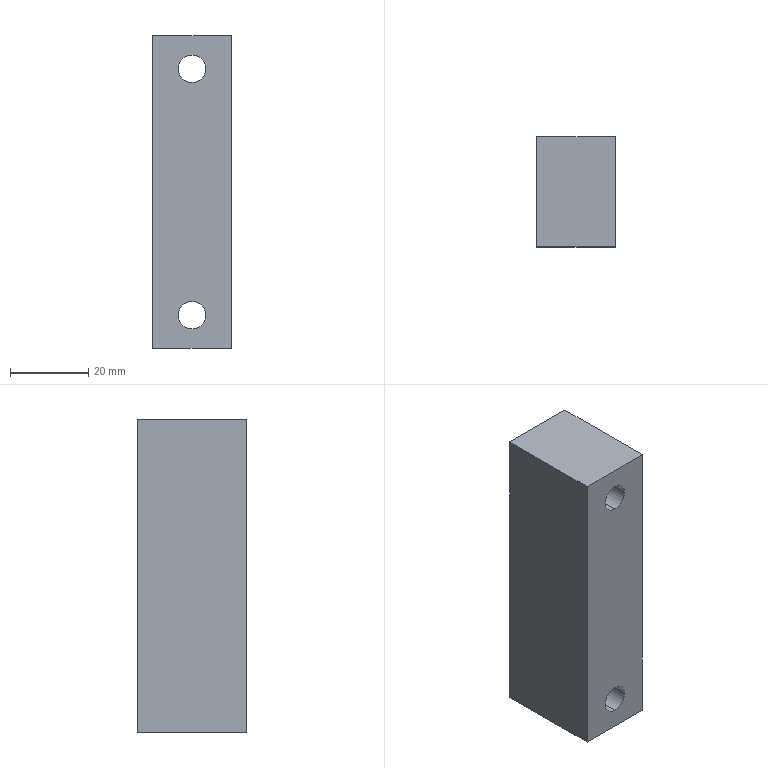Component | SolidWorks | BearingHeighteningSeat-1 | 1 solid | 10 faces | box 20 x 28 x 80 mm | volume 42645 mm3 | plane 6 | cylinder 4 | commonest cylinder face diameters 7 x4
build123d program:
from build123d import *

# Parameters (mm, degrees)
SKETCH1_W      = 80
SKETCH1_H      = 20
SKETCH1_R      = 3.5
EXTRUDE1_DEPTH = 28


with BuildPart() as part:
    # Sketch1 → Extrude1 (new body)
    with BuildSketch(Plane.XY):
        with Locations((-20.645, 10.76)):
            Rectangle(SKETCH1_W, SKETCH1_H)
        with Locations((-52.145, 10.76)):
            Circle(SKETCH1_R, mode=Mode.SUBTRACT)
        with Locations((10.855, 10.76)):
            Circle(SKETCH1_R, mode=Mode.SUBTRACT)
    extrude(amount=EXTRUDE1_DEPTH)


solid = part.part

# Placed as in the assembly
solid = solid.moved(Location((190.976, 153.983, 79.382), (90, 0, 90)))
STEP:
#1=COLOUR_RGB('',0.7922,0.8196,0.9333);
#2=FILL_AREA_STYLE_COLOUR('',#1);
#3=FILL_AREA_STYLE('',(#2));
#4=SURFACE_STYLE_FILL_AREA(#3);
#5=SURFACE_SIDE_STYLE('',(#4));
#6=SURFACE_STYLE_USAGE(.BOTH.,#5);
#7=PRESENTATION_STYLE_ASSIGNMENT((#6));
#8=CARTESIAN_POINT('',(7.095,6.062,3.415));
#9=VERTEX_POINT('',#8);
#10=CARTESIAN_POINT('',(7.095,6.062,3.69));
#11=VERTEX_POINT('',#10);
#12=CARTESIAN_POINT('',(7.095,6.062,3.553));
#13=DIRECTION('',(-0.,1.,-0.));
#14=DIRECTION('',(0.,0.,1.));
#15=AXIS2_PLACEMENT_3D('',#12,#13,#14);
#16=CIRCLE('',#15,0.1378);
#17=EDGE_CURVE('',#9,#11,#16,.T.);
#18=ORIENTED_EDGE('',*,*,#17,.T.);
#19=CARTESIAN_POINT('',(7.095,4.96,3.69));
#20=VERTEX_POINT('',#19);
#21=CARTESIAN_POINT('',(7.095,6.062,3.69));
#22=DIRECTION('',(0.,-1.,0.));
#23=VECTOR('',#22,39.37);
#24=LINE('',#21,#23);
#25=EDGE_CURVE('',#11,#20,#24,.T.);
#26=ORIENTED_EDGE('',*,*,#25,.T.);
#27=CARTESIAN_POINT('',(7.095,4.96,3.415));
#28=VERTEX_POINT('',#27);
#29=CARTESIAN_POINT('',(7.095,4.96,3.553));
#30=DIRECTION('',(-0.,1.,-0.));
#31=DIRECTION('',(0.,0.,1.));
#32=AXIS2_PLACEMENT_3D('',#29,#30,#31);
#33=CIRCLE('',#32,0.1378);
#34=EDGE_CURVE('',#28,#20,#33,.T.);
#35=ORIENTED_EDGE('',*,*,#34,.F.);
#36=CARTESIAN_POINT('',(7.095,6.062,3.415));
#37=DIRECTION('',(0.,-1.,0.));
#38=VECTOR('',#37,39.37);
#39=LINE('',#36,#38);
#40=EDGE_CURVE('',#9,#28,#39,.T.);
#41=ORIENTED_EDGE('',*,*,#40,.F.);
#42=EDGE_LOOP('',(#18,#26,#35,#41));
#43=FACE_OUTER_BOUND('',#42,.T.);
#44=CARTESIAN_POINT('',(7.095,6.062,3.553));
#45=DIRECTION('',(0.,-1.,0.));
#46=DIRECTION('',(0.,0.,-1.));
#47=AXIS2_PLACEMENT_3D('',#44,#45,#46);
#48=CYLINDRICAL_SURFACE('',#47,0.1378);
#49=ADVANCED_FACE('',(#43),#48,.F.);
#50=CARTESIAN_POINT('',(7.095,6.062,0.9345));
#51=VERTEX_POINT('',#50);
#52=CARTESIAN_POINT('',(7.095,6.062,1.21));
#53=VERTEX_POINT('',#52);
#54=CARTESIAN_POINT('',(7.095,6.062,1.072));
#55=DIRECTION('',(-0.,1.,-0.));
#56=DIRECTION('',(0.,0.,1.));
#57=AXIS2_PLACEMENT_3D('',#54,#55,#56);
#58=CIRCLE('',#57,0.1378);
#59=EDGE_CURVE('',#51,#53,#58,.T.);
#60=ORIENTED_EDGE('',*,*,#59,.T.);
#61=CARTESIAN_POINT('',(7.095,4.96,1.21));
#62=VERTEX_POINT('',#61);
#63=CARTESIAN_POINT('',(7.095,6.062,1.21));
#64=DIRECTION('',(0.,-1.,0.));
#65=VECTOR('',#64,39.37);
#66=LINE('',#63,#65);
#67=EDGE_CURVE('',#53,#62,#66,.T.);
#68=ORIENTED_EDGE('',*,*,#67,.T.);
#69=CARTESIAN_POINT('',(7.095,4.96,0.9345));
#70=VERTEX_POINT('',#69);
#71=CARTESIAN_POINT('',(7.095,4.96,1.072));
#72=DIRECTION('',(-0.,1.,-0.));
#73=DIRECTION('',(0.,0.,1.));
#74=AXIS2_PLACEMENT_3D('',#71,#72,#73);
#75=CIRCLE('',#74,0.1378);
#76=EDGE_CURVE('',#70,#62,#75,.T.);
#77=ORIENTED_EDGE('',*,*,#76,.F.);
#78=CARTESIAN_POINT('',(7.095,6.062,0.9345));
#79=DIRECTION('',(0.,-1.,0.));
#80=VECTOR('',#79,39.37);
#81=LINE('',#78,#80);
#82=EDGE_CURVE('',#51,#70,#81,.T.);
#83=ORIENTED_EDGE('',*,*,#82,.F.);
#84=EDGE_LOOP('',(#60,#68,#77,#83));
#85=FACE_OUTER_BOUND('',#84,.T.);
#86=CARTESIAN_POINT('',(7.095,6.062,1.072));
#87=DIRECTION('',(0.,-1.,0.));
#88=DIRECTION('',(0.,0.,-1.));
#89=AXIS2_PLACEMENT_3D('',#86,#87,#88);
#90=CYLINDRICAL_SURFACE('',#89,0.1378);
#91=ADVANCED_FACE('',(#85),#90,.F.);
#92=ORIENTED_EDGE('',*,*,#59,.F.);
#93=CARTESIAN_POINT('',(7.095,6.062,1.072));
#94=DIRECTION('',(-0.,1.,-0.));
#95=DIRECTION('',(0.,0.,1.));
#96=AXIS2_PLACEMENT_3D('',#93,#94,#95);
#97=CIRCLE('',#96,0.1378);
#98=EDGE_CURVE('',#53,#51,#97,.T.);
#99=ORIENTED_EDGE('',*,*,#98,.F.);
#100=EDGE_LOOP('',(#92,#99));
#101=FACE_BOUND('',#100,.T.);
#102=CARTESIAN_POINT('',(7.489,6.062,0.7377));
#103=VERTEX_POINT('',#102);
#104=CARTESIAN_POINT('',(6.701,6.062,0.7377));
#105=VERTEX_POINT('',#104);
#106=CARTESIAN_POINT('',(7.489,6.062,0.7377));
#107=DIRECTION('',(-1.,0.,0.));
#108=VECTOR('',#107,39.37);
#109=LINE('',#106,#108);
#110=EDGE_CURVE('',#103,#105,#109,.T.);
#111=ORIENTED_EDGE('',*,*,#110,.T.);
#112=CARTESIAN_POINT('',(6.701,6.062,3.887));
#113=VERTEX_POINT('',#112);
#114=CARTESIAN_POINT('',(6.701,6.062,0.7377));
#115=DIRECTION('',(-0.,0.,1.));
#116=VECTOR('',#115,39.37);
#117=LINE('',#114,#116);
#118=EDGE_CURVE('',#105,#113,#117,.T.);
#119=ORIENTED_EDGE('',*,*,#118,.T.);
#120=CARTESIAN_POINT('',(7.489,6.062,3.887));
#121=VERTEX_POINT('',#120);
#122=CARTESIAN_POINT('',(7.489,6.062,3.887));
#123=DIRECTION('',(1.,-0.,-0.));
#124=VECTOR('',#123,39.37);
#125=LINE('',#122,#124);
#126=EDGE_CURVE('',#113,#121,#125,.T.);
#127=ORIENTED_EDGE('',*,*,#126,.T.);
#128=CARTESIAN_POINT('',(7.489,6.062,0.7377));
#129=DIRECTION('',(0.,-0.,-1.));
#130=VECTOR('',#129,39.37);
#131=LINE('',#128,#130);
#132=EDGE_CURVE('',#121,#103,#131,.T.);
#133=ORIENTED_EDGE('',*,*,#132,.T.);
#134=EDGE_LOOP('',(#111,#119,#127,#133));
#135=FACE_OUTER_BOUND('',#134,.T.);
#136=ORIENTED_EDGE('',*,*,#17,.F.);
#137=CARTESIAN_POINT('',(7.095,6.062,3.553));
#138=DIRECTION('',(-0.,1.,-0.));
#139=DIRECTION('',(0.,0.,1.));
#140=AXIS2_PLACEMENT_3D('',#137,#138,#139);
#141=CIRCLE('',#140,0.1378);
#142=EDGE_CURVE('',#11,#9,#141,.T.);
#143=ORIENTED_EDGE('',*,*,#142,.F.);
#144=EDGE_LOOP('',(#136,#143));
#145=FACE_BOUND('',#144,.T.);
#146=CARTESIAN_POINT('',(6.701,6.062,0.7377));
#147=DIRECTION('',(-0.,1.,-0.));
#148=DIRECTION('',(-0.,0.,1.));
#149=AXIS2_PLACEMENT_3D('',#146,#147,#148);
#150=PLANE('',#149);
#151=ADVANCED_FACE('',(#101,#135,#145),#150,.T.);
#152=CARTESIAN_POINT('',(7.489,4.96,0.7377));
#153=VERTEX_POINT('',#152);
#154=CARTESIAN_POINT('',(6.701,4.96,0.7377));
#155=VERTEX_POINT('',#154);
#156=CARTESIAN_POINT('',(7.489,4.96,0.7377));
#157=DIRECTION('',(-1.,0.,0.));
#158=VECTOR('',#157,39.37);
#159=LINE('',#156,#158);
#160=EDGE_CURVE('',#153,#155,#159,.T.);
#161=ORIENTED_EDGE('',*,*,#160,.F.);
#162=CARTESIAN_POINT('',(7.489,4.96,3.887));
#163=VERTEX_POINT('',#162);
#164=CARTESIAN_POINT('',(7.489,4.96,0.7377));
#165=DIRECTION('',(0.,-0.,-1.));
#166=VECTOR('',#165,39.37);
#167=LINE('',#164,#166);
#168=EDGE_CURVE('',#163,#153,#167,.T.);
#169=ORIENTED_EDGE('',*,*,#168,.F.);
#170=CARTESIAN_POINT('',(6.701,4.96,3.887));
#171=VERTEX_POINT('',#170);
#172=CARTESIAN_POINT('',(7.489,4.96,3.887));
#173=DIRECTION('',(1.,-0.,-0.));
#174=VECTOR('',#173,39.37);
#175=LINE('',#172,#174);
#176=EDGE_CURVE('',#171,#163,#175,.T.);
#177=ORIENTED_EDGE('',*,*,#176,.F.);
#178=CARTESIAN_POINT('',(6.701,4.96,0.7377));
#179=DIRECTION('',(-0.,0.,1.));
#180=VECTOR('',#179,39.37);
#181=LINE('',#178,#180);
#182=EDGE_CURVE('',#155,#171,#181,.T.);
#183=ORIENTED_EDGE('',*,*,#182,.F.);
#184=EDGE_LOOP('',(#161,#169,#177,#183));
#185=FACE_OUTER_BOUND('',#184,.T.);
#186=ORIENTED_EDGE('',*,*,#76,.T.);
#187=CARTESIAN_POINT('',(7.095,4.96,1.072));
#188=DIRECTION('',(-0.,1.,-0.));
#189=DIRECTION('',(0.,0.,1.));
#190=AXIS2_PLACEMENT_3D('',#187,#188,#189);
#191=CIRCLE('',#190,0.1378);
#192=EDGE_CURVE('',#62,#70,#191,.T.);
#193=ORIENTED_EDGE('',*,*,#192,.T.);
#194=EDGE_LOOP('',(#186,#193));
#195=FACE_BOUND('',#194,.T.);
#196=ORIENTED_EDGE('',*,*,#34,.T.);
#197=CARTESIAN_POINT('',(7.095,4.96,3.553));
#198=DIRECTION('',(-0.,1.,-0.));
#199=DIRECTION('',(0.,0.,1.));
#200=AXIS2_PLACEMENT_3D('',#197,#198,#199);
#201=CIRCLE('',#200,0.1378);
#202=EDGE_CURVE('',#20,#28,#201,.T.);
#203=ORIENTED_EDGE('',*,*,#202,.T.);
#204=EDGE_LOOP('',(#196,#203));
#205=FACE_BOUND('',#204,.T.);
#206=CARTESIAN_POINT('',(6.701,4.96,0.7377));
#207=DIRECTION('',(-0.,1.,-0.));
#208=DIRECTION('',(-0.,0.,1.));
#209=AXIS2_PLACEMENT_3D('',#206,#207,#208);
#210=PLANE('',#209);
#211=ADVANCED_FACE('',(#185,#195,#205),#210,.F.);
#212=ORIENTED_EDGE('',*,*,#160,.T.);
#213=CARTESIAN_POINT('',(6.701,6.062,0.7377));
#214=DIRECTION('',(0.,-1.,0.));
#215=VECTOR('',#214,39.37);
#216=LINE('',#213,#215);
#217=EDGE_CURVE('',#105,#155,#216,.T.);
#218=ORIENTED_EDGE('',*,*,#217,.F.);
#219=ORIENTED_EDGE('',*,*,#110,.F.);
#220=CARTESIAN_POINT('',(7.489,6.062,0.7377));
#221=DIRECTION('',(0.,-1.,0.));
#222=VECTOR('',#221,39.37);
#223=LINE('',#220,#222);
#224=EDGE_CURVE('',#103,#153,#223,.T.);
#225=ORIENTED_EDGE('',*,*,#224,.T.);
#226=EDGE_LOOP('',(#212,#218,#219,#225));
#227=FACE_OUTER_BOUND('',#226,.T.);
#228=CARTESIAN_POINT('',(7.489,6.062,0.7377));
#229=DIRECTION('',(0.,0.,1.));
#230=DIRECTION('',(1.,-0.,-0.));
#231=AXIS2_PLACEMENT_3D('',#228,#229,#230);
#232=PLANE('',#231);
#233=ADVANCED_FACE('',(#227),#232,.F.);
#234=ORIENTED_EDGE('',*,*,#182,.T.);
#235=CARTESIAN_POINT('',(6.701,6.062,3.887));
#236=DIRECTION('',(0.,-1.,0.));
#237=VECTOR('',#236,39.37);
#238=LINE('',#235,#237);
#239=EDGE_CURVE('',#113,#171,#238,.T.);
#240=ORIENTED_EDGE('',*,*,#239,.F.);
#241=ORIENTED_EDGE('',*,*,#118,.F.);
#242=ORIENTED_EDGE('',*,*,#217,.T.);
#243=EDGE_LOOP('',(#234,#240,#241,#242));
#244=FACE_OUTER_BOUND('',#243,.T.);
#245=CARTESIAN_POINT('',(6.701,6.062,0.7377));
#246=DIRECTION('',(1.,0.,0.));
#247=DIRECTION('',(-0.,1.,-0.));
#248=AXIS2_PLACEMENT_3D('',#245,#246,#247);
#249=PLANE('',#248);
#250=ADVANCED_FACE('',(#244),#249,.F.);
#251=ORIENTED_EDGE('',*,*,#176,.T.);
#252=CARTESIAN_POINT('',(7.489,6.062,3.887));
#253=DIRECTION('',(0.,-1.,0.));
#254=VECTOR('',#253,39.37);
#255=LINE('',#252,#254);
#256=EDGE_CURVE('',#121,#163,#255,.T.);
#257=ORIENTED_EDGE('',*,*,#256,.F.);
#258=ORIENTED_EDGE('',*,*,#126,.F.);
#259=ORIENTED_EDGE('',*,*,#239,.T.);
#260=EDGE_LOOP('',(#251,#257,#258,#259));
#261=FACE_OUTER_BOUND('',#260,.T.);
#262=CARTESIAN_POINT('',(7.489,6.062,3.887));
#263=DIRECTION('',(-0.,-0.,-1.));
#264=DIRECTION('',(-1.,0.,0.));
#265=AXIS2_PLACEMENT_3D('',#262,#263,#264);
#266=PLANE('',#265);
#267=ADVANCED_FACE('',(#261),#266,.F.);
#268=ORIENTED_EDGE('',*,*,#168,.T.);
#269=ORIENTED_EDGE('',*,*,#224,.F.);
#270=ORIENTED_EDGE('',*,*,#132,.F.);
#271=ORIENTED_EDGE('',*,*,#256,.T.);
#272=EDGE_LOOP('',(#268,#269,#270,#271));
#273=FACE_OUTER_BOUND('',#272,.T.);
#274=CARTESIAN_POINT('',(7.489,6.062,0.7377));
#275=DIRECTION('',(-1.,-0.,-0.));
#276=DIRECTION('',(0.,-1.,0.));
#277=AXIS2_PLACEMENT_3D('',#274,#275,#276);
#278=PLANE('',#277);
#279=ADVANCED_FACE('',(#273),#278,.F.);
#280=ORIENTED_EDGE('',*,*,#67,.F.);
#281=ORIENTED_EDGE('',*,*,#98,.T.);
#282=ORIENTED_EDGE('',*,*,#82,.T.);
#283=ORIENTED_EDGE('',*,*,#192,.F.);
#284=EDGE_LOOP('',(#280,#281,#282,#283));
#285=FACE_OUTER_BOUND('',#284,.T.);
#286=CARTESIAN_POINT('',(7.095,6.062,1.072));
#287=DIRECTION('',(0.,-1.,0.));
#288=DIRECTION('',(0.,0.,-1.));
#289=AXIS2_PLACEMENT_3D('',#286,#287,#288);
#290=CYLINDRICAL_SURFACE('',#289,0.1378);
#291=ADVANCED_FACE('',(#285),#290,.F.);
#292=ORIENTED_EDGE('',*,*,#25,.F.);
#293=ORIENTED_EDGE('',*,*,#142,.T.);
#294=ORIENTED_EDGE('',*,*,#40,.T.);
#295=ORIENTED_EDGE('',*,*,#202,.F.);
#296=EDGE_LOOP('',(#292,#293,#294,#295));
#297=FACE_OUTER_BOUND('',#296,.T.);
#298=CARTESIAN_POINT('',(7.095,6.062,3.553));
#299=DIRECTION('',(0.,-1.,0.));
#300=DIRECTION('',(0.,0.,-1.));
#301=AXIS2_PLACEMENT_3D('',#298,#299,#300);
#302=CYLINDRICAL_SURFACE('',#301,0.1378);
#303=ADVANCED_FACE('',(#297),#302,.F.);
#304=CLOSED_SHELL('',(#49,#91,#151,#211,#233,#250,#267,#279,#291,#303));
#305=MANIFOLD_SOLID_BREP('',#304);
#306=STYLED_ITEM('',(#7),#305);
#307=(LENGTH_UNIT()NAMED_UNIT(*)SI_UNIT($,.METRE.));
#308=LENGTH_MEASURE_WITH_UNIT(LENGTH_MEASURE(0.0254),#307);
#309=DIMENSIONAL_EXPONENTS(1.,0.,0.,0.,0.,0.,0.);
#310=(CONVERSION_BASED_UNIT('',#308)LENGTH_UNIT()NAMED_UNIT(#309));
#311=UNCERTAINTY_MEASURE_WITH_UNIT(LENGTH_MEASURE(0.00001),#310,'','');
#312=(NAMED_UNIT(*)PLANE_ANGLE_UNIT()SI_UNIT($,.RADIAN.));
#313=(NAMED_UNIT(*)SI_UNIT($,.STERADIAN.)SOLID_ANGLE_UNIT());
#314=(GEOMETRIC_REPRESENTATION_CONTEXT(3)GLOBAL_UNCERTAINTY_ASSIGNED_CONTEXT((#311))GLOBAL_UNIT_ASSIGNED_CONTEXT((#310,#312,#313))REPRESENTATION_CONTEXT('',''));
#315=MECHANICAL_DESIGN_GEOMETRIC_PRESENTATION_REPRESENTATION('',(#306),#314);
#316=PRESENTATION_LAYER_ASSIGNMENT('','',(#306));
#317=CARTESIAN_POINT('',(0.,0.,0.));
#318=DIRECTION('',(0.,0.,1.));
#319=DIRECTION('',(1.,0.,0.));
#320=AXIS2_PLACEMENT_3D('',#317,#318,#319);
#321=(LENGTH_UNIT()NAMED_UNIT(*)SI_UNIT($,.METRE.));
#322=LENGTH_MEASURE_WITH_UNIT(LENGTH_MEASURE(0.0254),#321);
#323=DIMENSIONAL_EXPONENTS(1.,0.,0.,0.,0.,0.,0.);
#324=(CONVERSION_BASED_UNIT('',#322)LENGTH_UNIT()NAMED_UNIT(#323));
#325=UNCERTAINTY_MEASURE_WITH_UNIT(LENGTH_MEASURE(0.00001),#324,'','');
#326=(NAMED_UNIT(*)PLANE_ANGLE_UNIT()SI_UNIT($,.RADIAN.));
#327=(NAMED_UNIT(*)SI_UNIT($,.STERADIAN.)SOLID_ANGLE_UNIT());
#328=(GEOMETRIC_REPRESENTATION_CONTEXT(3)GLOBAL_UNCERTAINTY_ASSIGNED_CONTEXT((#325))GLOBAL_UNIT_ASSIGNED_CONTEXT((#324,#326,#327))REPRESENTATION_CONTEXT('',''));
#329=ADVANCED_BREP_SHAPE_REPRESENTATION('',(#305,#320),#328);